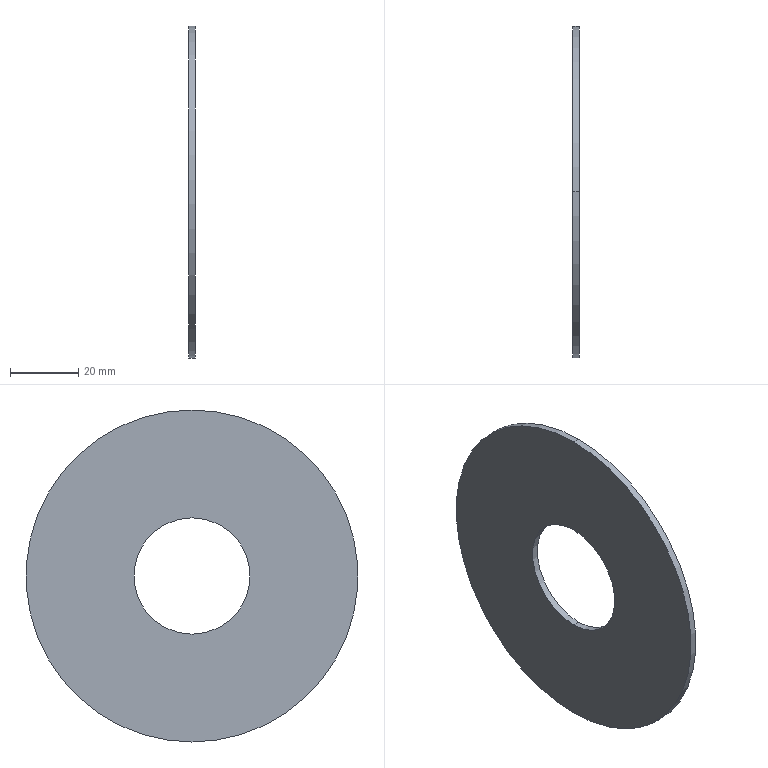Component | SolidWorks | SealRing3-1 | 1 solid | 6 faces | box 2 x 97 x 97 mm | volume 12964 mm3 | cylinder 4 | plane 2 | commonest cylinder face diameters 34 x2 97 x2
build123d program:
from build123d import *

# Parameters (mm, degrees)
SKETCH2_R           = 48.5
SKETCH2_R_2         = 17
BOSS_EXTRUDE1_DEPTH = 2


with BuildPart() as part:
    # Sketch2 → Boss-Extrude1 (new body)
    with BuildSketch(Plane(origin=(0, 0, 0), x_dir=(0, 0, -1), z_dir=(1, 0, 0))):
        Circle(SKETCH2_R)
        Circle(SKETCH2_R_2, mode=Mode.SUBTRACT)
    extrude(amount=BOSS_EXTRUDE1_DEPTH)


solid = part.part

# Placed as in the assembly
solid = solid.moved(Location((-43.66, 0, 0), (0, 0, 0)))
STEP:
#1=CARTESIAN_POINT('',(-1.64,-0.,0.6693));
#2=VERTEX_POINT('',#1);
#3=CARTESIAN_POINT('',(-1.64,-0.,-0.6693));
#4=VERTEX_POINT('',#3);
#5=CARTESIAN_POINT('',(-1.64,-0.,0.));
#6=DIRECTION('',(1.,0.,0.));
#7=DIRECTION('',(0.,0.,-1.));
#8=AXIS2_PLACEMENT_3D('',#5,#6,#7);
#9=CIRCLE('',#8,0.6693);
#10=EDGE_CURVE('',#2,#4,#9,.T.);
#11=ORIENTED_EDGE('',*,*,#10,.T.);
#12=CARTESIAN_POINT('',(-1.719,-0.,-0.6693));
#13=VERTEX_POINT('',#12);
#14=CARTESIAN_POINT('',(-1.64,-0.,-0.6693));
#15=DIRECTION('',(-1.,0.,0.));
#16=VECTOR('',#15,39.37);
#17=LINE('',#14,#16);
#18=EDGE_CURVE('',#4,#13,#17,.T.);
#19=ORIENTED_EDGE('',*,*,#18,.T.);
#20=CARTESIAN_POINT('',(-1.719,-0.,0.6693));
#21=VERTEX_POINT('',#20);
#22=CARTESIAN_POINT('',(-1.719,-0.,0.));
#23=DIRECTION('',(1.,0.,0.));
#24=DIRECTION('',(0.,0.,-1.));
#25=AXIS2_PLACEMENT_3D('',#22,#23,#24);
#26=CIRCLE('',#25,0.6693);
#27=EDGE_CURVE('',#21,#13,#26,.T.);
#28=ORIENTED_EDGE('',*,*,#27,.F.);
#29=CARTESIAN_POINT('',(-1.64,-0.,0.6693));
#30=DIRECTION('',(-1.,0.,0.));
#31=VECTOR('',#30,39.37);
#32=LINE('',#29,#31);
#33=EDGE_CURVE('',#2,#21,#32,.T.);
#34=ORIENTED_EDGE('',*,*,#33,.F.);
#35=EDGE_LOOP('',(#11,#19,#28,#34));
#36=FACE_OUTER_BOUND('',#35,.T.);
#37=CARTESIAN_POINT('',(-1.64,-0.,0.));
#38=DIRECTION('',(-1.,0.,0.));
#39=DIRECTION('',(0.,0.,1.));
#40=AXIS2_PLACEMENT_3D('',#37,#38,#39);
#41=CYLINDRICAL_SURFACE('',#40,0.6693);
#42=ADVANCED_FACE('',(#36),#41,.F.);
#43=CARTESIAN_POINT('',(-1.64,-0.,-1.909));
#44=VERTEX_POINT('',#43);
#45=CARTESIAN_POINT('',(-1.64,-0.,1.909));
#46=VERTEX_POINT('',#45);
#47=CARTESIAN_POINT('',(-1.64,-0.,0.));
#48=DIRECTION('',(1.,0.,0.));
#49=DIRECTION('',(0.,0.,-1.));
#50=AXIS2_PLACEMENT_3D('',#47,#48,#49);
#51=CIRCLE('',#50,1.909);
#52=EDGE_CURVE('',#44,#46,#51,.T.);
#53=ORIENTED_EDGE('',*,*,#52,.F.);
#54=CARTESIAN_POINT('',(-1.719,-0.,-1.909));
#55=VERTEX_POINT('',#54);
#56=CARTESIAN_POINT('',(-1.64,-0.,-1.909));
#57=DIRECTION('',(-1.,0.,0.));
#58=VECTOR('',#57,39.37);
#59=LINE('',#56,#58);
#60=EDGE_CURVE('',#44,#55,#59,.T.);
#61=ORIENTED_EDGE('',*,*,#60,.T.);
#62=CARTESIAN_POINT('',(-1.719,-0.,1.909));
#63=VERTEX_POINT('',#62);
#64=CARTESIAN_POINT('',(-1.719,-0.,0.));
#65=DIRECTION('',(1.,0.,0.));
#66=DIRECTION('',(0.,0.,-1.));
#67=AXIS2_PLACEMENT_3D('',#64,#65,#66);
#68=CIRCLE('',#67,1.909);
#69=EDGE_CURVE('',#55,#63,#68,.T.);
#70=ORIENTED_EDGE('',*,*,#69,.T.);
#71=CARTESIAN_POINT('',(-1.64,-0.,1.909));
#72=DIRECTION('',(-1.,0.,0.));
#73=VECTOR('',#72,39.37);
#74=LINE('',#71,#73);
#75=EDGE_CURVE('',#46,#63,#74,.T.);
#76=ORIENTED_EDGE('',*,*,#75,.F.);
#77=EDGE_LOOP('',(#53,#61,#70,#76));
#78=FACE_OUTER_BOUND('',#77,.T.);
#79=CARTESIAN_POINT('',(-1.64,-0.,0.));
#80=DIRECTION('',(-1.,0.,0.));
#81=DIRECTION('',(0.,0.,1.));
#82=AXIS2_PLACEMENT_3D('',#79,#80,#81);
#83=CYLINDRICAL_SURFACE('',#82,1.909);
#84=ADVANCED_FACE('',(#78),#83,.T.);
#85=CARTESIAN_POINT('',(-1.64,-0.,0.));
#86=DIRECTION('',(1.,0.,0.));
#87=DIRECTION('',(0.,0.,-1.));
#88=AXIS2_PLACEMENT_3D('',#85,#86,#87);
#89=CIRCLE('',#88,1.909);
#90=EDGE_CURVE('',#46,#44,#89,.T.);
#91=ORIENTED_EDGE('',*,*,#90,.T.);
#92=ORIENTED_EDGE('',*,*,#52,.T.);
#93=EDGE_LOOP('',(#91,#92));
#94=FACE_OUTER_BOUND('',#93,.T.);
#95=ORIENTED_EDGE('',*,*,#10,.F.);
#96=CARTESIAN_POINT('',(-1.64,-0.,0.));
#97=DIRECTION('',(1.,0.,0.));
#98=DIRECTION('',(0.,0.,-1.));
#99=AXIS2_PLACEMENT_3D('',#96,#97,#98);
#100=CIRCLE('',#99,0.6693);
#101=EDGE_CURVE('',#4,#2,#100,.T.);
#102=ORIENTED_EDGE('',*,*,#101,.F.);
#103=EDGE_LOOP('',(#95,#102));
#104=FACE_BOUND('',#103,.T.);
#105=CARTESIAN_POINT('',(-1.64,-0.,0.));
#106=DIRECTION('',(1.,0.,0.));
#107=DIRECTION('',(0.,0.,-1.));
#108=AXIS2_PLACEMENT_3D('',#105,#106,#107);
#109=PLANE('',#108);
#110=ADVANCED_FACE('',(#94,#104),#109,.T.);
#111=CARTESIAN_POINT('',(-1.719,-0.,0.));
#112=DIRECTION('',(1.,0.,0.));
#113=DIRECTION('',(0.,0.,-1.));
#114=AXIS2_PLACEMENT_3D('',#111,#112,#113);
#115=CIRCLE('',#114,1.909);
#116=EDGE_CURVE('',#63,#55,#115,.T.);
#117=ORIENTED_EDGE('',*,*,#116,.F.);
#118=ORIENTED_EDGE('',*,*,#69,.F.);
#119=EDGE_LOOP('',(#117,#118));
#120=FACE_OUTER_BOUND('',#119,.T.);
#121=ORIENTED_EDGE('',*,*,#27,.T.);
#122=CARTESIAN_POINT('',(-1.719,-0.,0.));
#123=DIRECTION('',(1.,0.,0.));
#124=DIRECTION('',(0.,0.,-1.));
#125=AXIS2_PLACEMENT_3D('',#122,#123,#124);
#126=CIRCLE('',#125,0.6693);
#127=EDGE_CURVE('',#13,#21,#126,.T.);
#128=ORIENTED_EDGE('',*,*,#127,.T.);
#129=EDGE_LOOP('',(#121,#128));
#130=FACE_BOUND('',#129,.T.);
#131=CARTESIAN_POINT('',(-1.719,-0.,0.));
#132=DIRECTION('',(1.,0.,0.));
#133=DIRECTION('',(0.,0.,-1.));
#134=AXIS2_PLACEMENT_3D('',#131,#132,#133);
#135=PLANE('',#134);
#136=ADVANCED_FACE('',(#120,#130),#135,.F.);
#137=ORIENTED_EDGE('',*,*,#60,.F.);
#138=ORIENTED_EDGE('',*,*,#90,.F.);
#139=ORIENTED_EDGE('',*,*,#75,.T.);
#140=ORIENTED_EDGE('',*,*,#116,.T.);
#141=EDGE_LOOP('',(#137,#138,#139,#140));
#142=FACE_OUTER_BOUND('',#141,.T.);
#143=CARTESIAN_POINT('',(-1.64,-0.,0.));
#144=DIRECTION('',(-1.,0.,0.));
#145=DIRECTION('',(0.,0.,1.));
#146=AXIS2_PLACEMENT_3D('',#143,#144,#145);
#147=CYLINDRICAL_SURFACE('',#146,1.909);
#148=ADVANCED_FACE('',(#142),#147,.T.);
#149=ORIENTED_EDGE('',*,*,#18,.F.);
#150=ORIENTED_EDGE('',*,*,#101,.T.);
#151=ORIENTED_EDGE('',*,*,#33,.T.);
#152=ORIENTED_EDGE('',*,*,#127,.F.);
#153=EDGE_LOOP('',(#149,#150,#151,#152));
#154=FACE_OUTER_BOUND('',#153,.T.);
#155=CARTESIAN_POINT('',(-1.64,-0.,0.));
#156=DIRECTION('',(-1.,0.,0.));
#157=DIRECTION('',(0.,0.,1.));
#158=AXIS2_PLACEMENT_3D('',#155,#156,#157);
#159=CYLINDRICAL_SURFACE('',#158,0.6693);
#160=ADVANCED_FACE('',(#154),#159,.F.);
#161=CLOSED_SHELL('',(#42,#84,#110,#136,#148,#160));
#162=MANIFOLD_SOLID_BREP('',#161);
#163=CARTESIAN_POINT('',(0.,0.,0.));
#164=DIRECTION('',(0.,0.,1.));
#165=DIRECTION('',(1.,0.,0.));
#166=AXIS2_PLACEMENT_3D('',#163,#164,#165);
#167=(LENGTH_UNIT()NAMED_UNIT(*)SI_UNIT($,.METRE.));
#168=LENGTH_MEASURE_WITH_UNIT(LENGTH_MEASURE(0.0254),#167);
#169=DIMENSIONAL_EXPONENTS(1.,0.,0.,0.,0.,0.,0.);
#170=(CONVERSION_BASED_UNIT('',#168)LENGTH_UNIT()NAMED_UNIT(#169));
#171=UNCERTAINTY_MEASURE_WITH_UNIT(LENGTH_MEASURE(0.00001),#170,'','');
#172=(NAMED_UNIT(*)PLANE_ANGLE_UNIT()SI_UNIT($,.RADIAN.));
#173=(NAMED_UNIT(*)SI_UNIT($,.STERADIAN.)SOLID_ANGLE_UNIT());
#174=(GEOMETRIC_REPRESENTATION_CONTEXT(3)GLOBAL_UNCERTAINTY_ASSIGNED_CONTEXT((#171))GLOBAL_UNIT_ASSIGNED_CONTEXT((#170,#172,#173))REPRESENTATION_CONTEXT('',''));
#175=ADVANCED_BREP_SHAPE_REPRESENTATION('',(#162,#166),#174);
#176=COLOUR_RGB('',0.7922,0.8196,0.9333);
#177=FILL_AREA_STYLE_COLOUR('',#176);
#178=FILL_AREA_STYLE('',(#177));
#179=SURFACE_STYLE_FILL_AREA(#178);
#180=SURFACE_SIDE_STYLE('',(#179));
#181=SURFACE_STYLE_USAGE(.BOTH.,#180);
#182=PRESENTATION_STYLE_ASSIGNMENT((#181));
#183=STYLED_ITEM('',(#182),#162);
#184=(LENGTH_UNIT()NAMED_UNIT(*)SI_UNIT($,.METRE.));
#185=LENGTH_MEASURE_WITH_UNIT(LENGTH_MEASURE(0.0254),#184);
#186=DIMENSIONAL_EXPONENTS(1.,0.,0.,0.,0.,0.,0.);
#187=(CONVERSION_BASED_UNIT('',#185)LENGTH_UNIT()NAMED_UNIT(#186));
#188=UNCERTAINTY_MEASURE_WITH_UNIT(LENGTH_MEASURE(0.00001),#187,'','');
#189=(NAMED_UNIT(*)PLANE_ANGLE_UNIT()SI_UNIT($,.RADIAN.));
#190=(NAMED_UNIT(*)SI_UNIT($,.STERADIAN.)SOLID_ANGLE_UNIT());
#191=(GEOMETRIC_REPRESENTATION_CONTEXT(3)GLOBAL_UNCERTAINTY_ASSIGNED_CONTEXT((#188))GLOBAL_UNIT_ASSIGNED_CONTEXT((#187,#189,#190))REPRESENTATION_CONTEXT('',''));
#192=MECHANICAL_DESIGN_GEOMETRIC_PRESENTATION_REPRESENTATION('',(#183),#191);
#193=PRESENTATION_LAYER_ASSIGNMENT('','',(#183));